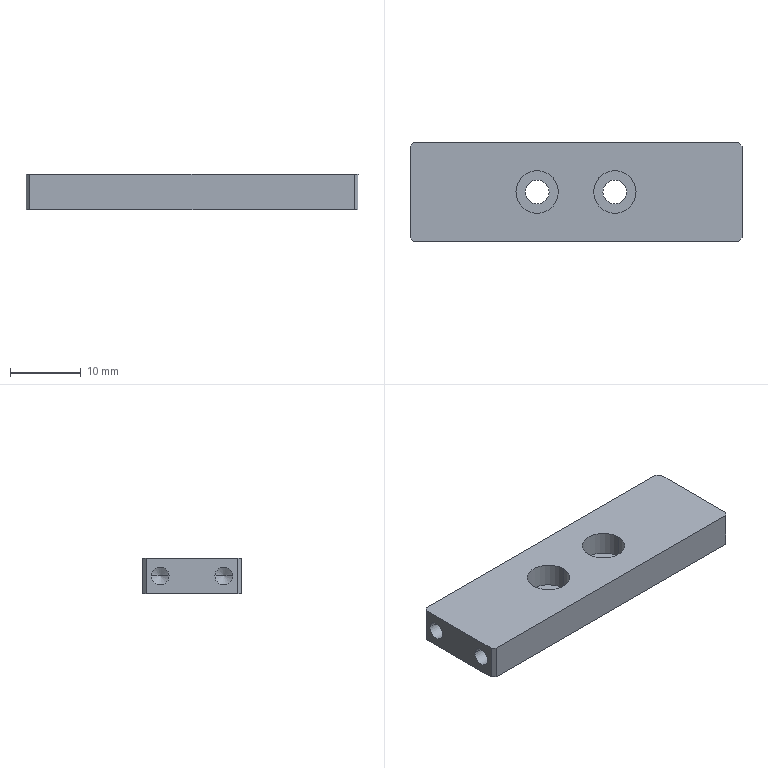Component | SolidWorks | F01AE00111-A5207-1 | 1 solid | 36 faces | box 47 x 14 x 5 mm | volume 2924 mm3 | cylinder 16 | plane 12 | cone 8 | commonest cylinder face diameters 2.5 x8 6 x4 3.4 x4
build123d program:
from build123d import *

# Parameters (mm, degrees)
SKETCH2_W                                            = 14
SKETCH2_H                                            = 5
BOSS_EXTRUDE1_DEPTH                                  = 23.5
HOLE_SIZE_ACCORDING_TO_THE_TYPE_OF_HEXAG_D           = 3.4
HOLE_SIZE_ACCORDING_TO_THE_TYPE_OF_HEXAG_CBORE_D     = 6
HOLE_SIZE_ACCORDING_TO_THE_TYPE_OF_HEXAG_CBORE_DEPTH = 3.4
M3_TAPPED_HOLE1_AT_2_COUNT                           = 2
M3_TAPPED_HOLE1_AT_2_PITCH                           = 9
CHAMFER1_SIZE                                        = 0.5


with BuildPart() as part:
    # Sketch2 → Boss-Extrude1 (new, symmetric)
    with BuildSketch(Plane.XY):
        with Locations((-7, 2.5)):
            Rectangle(SKETCH2_W, SKETCH2_H)
    extrude(amount=BOSS_EXTRUDE1_DEPTH, both=True)

    # Hole size according to the type of hexag (through all)
    with Locations(Plane(origin=(0, 5, 0), x_dir=(1, 0, 0), z_dir=(0, 1, 0))):
        with Locations((-7, 5.5), (-7, -5.5)):
            CounterBoreHole(HOLE_SIZE_ACCORDING_TO_THE_TYPE_OF_HEXAG_D / 2, HOLE_SIZE_ACCORDING_TO_THE_TYPE_OF_HEXAG_CBORE_D / 2, HOLE_SIZE_ACCORDING_TO_THE_TYPE_OF_HEXAG_CBORE_DEPTH)

    # Sketch7 → M3 Tapped Hole1 (revolve, cut)
    with BuildSketch(Plane(origin=(-2.5, 2.5, 23.5), x_dir=(0, -1, 0), z_dir=(1, 0, 0))):
        Polygon((0, 0), (0, 7.751), (1.25, 7), (1.25, 0), align=None)
    m3_tapped_hole1 = revolve(axis=Axis((-2.5, 2.5, 29.85), (0, 0, -1)), mode=Mode.SUBTRACT)

    # M3 Tapped Hole1 at 2: M3 Tapped Hole1 ×2
    with Locations(*[(-i * M3_TAPPED_HOLE1_AT_2_PITCH, 0, 0) for i in range(1, M3_TAPPED_HOLE1_AT_2_COUNT)]):
        add(m3_tapped_hole1, mode=Mode.SUBTRACT)

    # Mirror1: M3 Tapped Hole1 across plane
    add(m3_tapped_hole1.mirror(Plane.XY), mode=Mode.SUBTRACT)

    # Mirror1 copy 1 sketch → Mirror1 copy 1 (revolve, cut)
    with BuildSketch(Plane(origin=(-11.5, 2.5, -23.5), x_dir=(0, -1, 0), z_dir=(1, 0, 0))):
        Polygon((0, 0), (0, -7.751), (1.25, -7), (1.25, 0), align=None)
    revolve(axis=Axis((-11.5, 2.5, -29.85), (0, 0, -1)), mode=Mode.SUBTRACT)

    # Chamfer1
    chamfer1_edges = [part.edges().sort_by_distance(p)[0] for p in [
        (-14, 2.5, 23.5),
        (0, 2.5, 23.5),
        (-14, 2.5, -23.5),
        (0, 2.5, -23.5),
    ]]
    chamfer(chamfer1_edges, length=CHAMFER1_SIZE)


solid = part.part

# Placed as in the assembly
solid = solid.moved(Location((-17.181, -124.273, -285.979), (90, -90, 0)))
STEP:
#1=COLOUR_RGB('',0.7922,0.8196,0.9333);
#2=FILL_AREA_STYLE_COLOUR('',#1);
#3=FILL_AREA_STYLE('',(#2));
#4=SURFACE_STYLE_FILL_AREA(#3);
#5=SURFACE_SIDE_STYLE('',(#4));
#6=SURFACE_STYLE_USAGE(.BOTH.,#5);
#7=PRESENTATION_STYLE_ASSIGNMENT((#6));
#8=CARTESIAN_POINT('',(-0.0268,-4.489,-11.161));
#9=VERTEX_POINT('',#8);
#10=CARTESIAN_POINT('',(-0.0268,-4.391,-11.161));
#11=VERTEX_POINT('',#10);
#12=CARTESIAN_POINT('',(-0.0268,-4.44,-11.161));
#13=DIRECTION('',(1.,-0.,-0.));
#14=DIRECTION('',(0.,1.,0.));
#15=AXIS2_PLACEMENT_3D('',#12,#13,#14);
#16=CIRCLE('',#15,0.04921);
#17=EDGE_CURVE('',#9,#11,#16,.T.);
#18=ORIENTED_EDGE('',*,*,#17,.F.);
#19=CARTESIAN_POINT('',(0.2488,-4.489,-11.161));
#20=VERTEX_POINT('',#19);
#21=CARTESIAN_POINT('',(0.2488,-4.489,-11.161));
#22=DIRECTION('',(1.,-0.,-0.));
#23=VECTOR('',#22,39.37);
#24=LINE('',#21,#23);
#25=EDGE_CURVE('',#9,#20,#24,.T.);
#26=ORIENTED_EDGE('',*,*,#25,.T.);
#27=CARTESIAN_POINT('',(0.2488,-4.391,-11.161));
#28=VERTEX_POINT('',#27);
#29=CARTESIAN_POINT('',(0.2488,-4.44,-11.161));
#30=DIRECTION('',(1.,-0.,-0.));
#31=DIRECTION('',(0.,1.,0.));
#32=AXIS2_PLACEMENT_3D('',#29,#30,#31);
#33=CIRCLE('',#32,0.04921);
#34=EDGE_CURVE('',#20,#28,#33,.T.);
#35=ORIENTED_EDGE('',*,*,#34,.T.);
#36=CARTESIAN_POINT('',(0.2488,-4.391,-11.161));
#37=DIRECTION('',(1.,-0.,-0.));
#38=VECTOR('',#37,39.37);
#39=LINE('',#36,#38);
#40=EDGE_CURVE('',#11,#28,#39,.T.);
#41=ORIENTED_EDGE('',*,*,#40,.F.);
#42=EDGE_LOOP('',(#18,#26,#35,#41));
#43=FACE_OUTER_BOUND('',#42,.T.);
#44=CARTESIAN_POINT('',(0.2488,-4.44,-11.161));
#45=DIRECTION('',(1.,-0.,-0.));
#46=DIRECTION('',(0.,1.,0.));
#47=AXIS2_PLACEMENT_3D('',#44,#45,#46);
#48=CYLINDRICAL_SURFACE('',#47,0.04921);
#49=ADVANCED_FACE('',(#43),#48,.F.);
#50=CARTESIAN_POINT('',(-0.05637,-4.44,-11.161));
#51=VERTEX_POINT('',#50);
#52=CARTESIAN_POINT('',(-0.0268,-4.391,-11.161));
#53=DIRECTION('',(0.515,0.8572,-0.));
#54=VECTOR('',#53,39.37);
#55=LINE('',#52,#54);
#56=EDGE_CURVE('',#51,#11,#55,.T.);
#57=ORIENTED_EDGE('',*,*,#56,.F.);
#58=CARTESIAN_POINT('',(-0.0268,-4.489,-11.161));
#59=DIRECTION('',(0.515,-0.8572,-0.));
#60=VECTOR('',#59,39.37);
#61=LINE('',#58,#60);
#62=EDGE_CURVE('',#51,#9,#61,.T.);
#63=ORIENTED_EDGE('',*,*,#62,.T.);
#64=ORIENTED_EDGE('',*,*,#17,.T.);
#65=EDGE_LOOP('',(#57,#63,#64));
#66=FACE_OUTER_BOUND('',#65,.T.);
#67=CARTESIAN_POINT('',(-0.0268,-4.44,-11.161));
#68=DIRECTION('',(1.,-0.,-0.));
#69=DIRECTION('',(0.,1.,0.));
#70=AXIS2_PLACEMENT_3D('',#67,#68,#69);
#71=CONICAL_SURFACE('',#70,0.04921,1.03);
#72=ADVANCED_FACE('',(#66),#71,.F.);
#73=CARTESIAN_POINT('',(-0.0268,-4.843,-11.161));
#74=VERTEX_POINT('',#73);
#75=CARTESIAN_POINT('',(-0.0268,-4.745,-11.161));
#76=VERTEX_POINT('',#75);
#77=CARTESIAN_POINT('',(-0.0268,-4.794,-11.161));
#78=DIRECTION('',(1.,-0.,-0.));
#79=DIRECTION('',(0.,1.,0.));
#80=AXIS2_PLACEMENT_3D('',#77,#78,#79);
#81=CIRCLE('',#80,0.04921);
#82=EDGE_CURVE('',#74,#76,#81,.T.);
#83=ORIENTED_EDGE('',*,*,#82,.F.);
#84=CARTESIAN_POINT('',(0.2488,-4.843,-11.161));
#85=VERTEX_POINT('',#84);
#86=CARTESIAN_POINT('',(0.2488,-4.843,-11.161));
#87=DIRECTION('',(1.,-0.,-0.));
#88=VECTOR('',#87,39.37);
#89=LINE('',#86,#88);
#90=EDGE_CURVE('',#74,#85,#89,.T.);
#91=ORIENTED_EDGE('',*,*,#90,.T.);
#92=CARTESIAN_POINT('',(0.2488,-4.745,-11.161));
#93=VERTEX_POINT('',#92);
#94=CARTESIAN_POINT('',(0.2488,-4.794,-11.161));
#95=DIRECTION('',(1.,-0.,-0.));
#96=DIRECTION('',(0.,1.,0.));
#97=AXIS2_PLACEMENT_3D('',#94,#95,#96);
#98=CIRCLE('',#97,0.04921);
#99=EDGE_CURVE('',#85,#93,#98,.T.);
#100=ORIENTED_EDGE('',*,*,#99,.T.);
#101=CARTESIAN_POINT('',(0.2488,-4.745,-11.161));
#102=DIRECTION('',(1.,-0.,-0.));
#103=VECTOR('',#102,39.37);
#104=LINE('',#101,#103);
#105=EDGE_CURVE('',#76,#93,#104,.T.);
#106=ORIENTED_EDGE('',*,*,#105,.F.);
#107=EDGE_LOOP('',(#83,#91,#100,#106));
#108=FACE_OUTER_BOUND('',#107,.T.);
#109=CARTESIAN_POINT('',(0.2488,-4.794,-11.161));
#110=DIRECTION('',(1.,-0.,-0.));
#111=DIRECTION('',(0.,1.,0.));
#112=AXIS2_PLACEMENT_3D('',#109,#110,#111);
#113=CYLINDRICAL_SURFACE('',#112,0.04921);
#114=ADVANCED_FACE('',(#108),#113,.F.);
#115=CARTESIAN_POINT('',(-0.05637,-4.794,-11.161));
#116=VERTEX_POINT('',#115);
#117=CARTESIAN_POINT('',(-0.0268,-4.745,-11.161));
#118=DIRECTION('',(0.515,0.8572,-0.));
#119=VECTOR('',#118,39.37);
#120=LINE('',#117,#119);
#121=EDGE_CURVE('',#116,#76,#120,.T.);
#122=ORIENTED_EDGE('',*,*,#121,.F.);
#123=CARTESIAN_POINT('',(-0.0268,-4.843,-11.161));
#124=DIRECTION('',(0.515,-0.8572,-0.));
#125=VECTOR('',#124,39.37);
#126=LINE('',#123,#125);
#127=EDGE_CURVE('',#116,#74,#126,.T.);
#128=ORIENTED_EDGE('',*,*,#127,.T.);
#129=ORIENTED_EDGE('',*,*,#82,.T.);
#130=EDGE_LOOP('',(#122,#128,#129));
#131=FACE_OUTER_BOUND('',#130,.T.);
#132=CARTESIAN_POINT('',(-0.0268,-4.794,-11.161));
#133=DIRECTION('',(1.,-0.,-0.));
#134=DIRECTION('',(0.,1.,0.));
#135=AXIS2_PLACEMENT_3D('',#132,#133,#134);
#136=CONICAL_SURFACE('',#135,0.04921,1.03);
#137=ADVANCED_FACE('',(#131),#136,.F.);
#138=CARTESIAN_POINT('',(-1.326,-4.391,-11.161));
#139=VERTEX_POINT('',#138);
#140=CARTESIAN_POINT('',(-1.326,-4.489,-11.161));
#141=VERTEX_POINT('',#140);
#142=CARTESIAN_POINT('',(-1.326,-4.44,-11.161));
#143=DIRECTION('',(-1.,0.,0.));
#144=DIRECTION('',(0.,-1.,0.));
#145=AXIS2_PLACEMENT_3D('',#142,#143,#144);
#146=CIRCLE('',#145,0.04921);
#147=EDGE_CURVE('',#139,#141,#146,.T.);
#148=ORIENTED_EDGE('',*,*,#147,.F.);
#149=CARTESIAN_POINT('',(-1.602,-4.391,-11.161));
#150=VERTEX_POINT('',#149);
#151=CARTESIAN_POINT('',(-1.602,-4.391,-11.161));
#152=DIRECTION('',(-1.,0.,0.));
#153=VECTOR('',#152,39.37);
#154=LINE('',#151,#153);
#155=EDGE_CURVE('',#139,#150,#154,.T.);
#156=ORIENTED_EDGE('',*,*,#155,.T.);
#157=CARTESIAN_POINT('',(-1.602,-4.489,-11.161));
#158=VERTEX_POINT('',#157);
#159=CARTESIAN_POINT('',(-1.602,-4.44,-11.161));
#160=DIRECTION('',(-1.,0.,0.));
#161=DIRECTION('',(0.,-1.,0.));
#162=AXIS2_PLACEMENT_3D('',#159,#160,#161);
#163=CIRCLE('',#162,0.04921);
#164=EDGE_CURVE('',#150,#158,#163,.T.);
#165=ORIENTED_EDGE('',*,*,#164,.T.);
#166=CARTESIAN_POINT('',(-1.602,-4.489,-11.161));
#167=DIRECTION('',(-1.,0.,0.));
#168=VECTOR('',#167,39.37);
#169=LINE('',#166,#168);
#170=EDGE_CURVE('',#141,#158,#169,.T.);
#171=ORIENTED_EDGE('',*,*,#170,.F.);
#172=EDGE_LOOP('',(#148,#156,#165,#171));
#173=FACE_OUTER_BOUND('',#172,.T.);
#174=CARTESIAN_POINT('',(-1.602,-4.44,-11.161));
#175=DIRECTION('',(-1.,0.,0.));
#176=DIRECTION('',(0.,-1.,0.));
#177=AXIS2_PLACEMENT_3D('',#174,#175,#176);
#178=CYLINDRICAL_SURFACE('',#177,0.04921);
#179=ADVANCED_FACE('',(#173),#178,.F.);
#180=CARTESIAN_POINT('',(-1.296,-4.44,-11.161));
#181=VERTEX_POINT('',#180);
#182=CARTESIAN_POINT('',(-1.326,-4.489,-11.161));
#183=DIRECTION('',(-0.515,-0.8572,0.));
#184=VECTOR('',#183,39.37);
#185=LINE('',#182,#184);
#186=EDGE_CURVE('',#181,#141,#185,.T.);
#187=ORIENTED_EDGE('',*,*,#186,.F.);
#188=CARTESIAN_POINT('',(-1.326,-4.391,-11.161));
#189=DIRECTION('',(-0.515,0.8572,0.));
#190=VECTOR('',#189,39.37);
#191=LINE('',#188,#190);
#192=EDGE_CURVE('',#181,#139,#191,.T.);
#193=ORIENTED_EDGE('',*,*,#192,.T.);
#194=ORIENTED_EDGE('',*,*,#147,.T.);
#195=EDGE_LOOP('',(#187,#193,#194));
#196=FACE_OUTER_BOUND('',#195,.T.);
#197=CARTESIAN_POINT('',(-1.326,-4.44,-11.161));
#198=DIRECTION('',(-1.,0.,0.));
#199=DIRECTION('',(0.,-1.,0.));
#200=AXIS2_PLACEMENT_3D('',#197,#198,#199);
#201=CONICAL_SURFACE('',#200,0.04921,1.03);
#202=ADVANCED_FACE('',(#196),#201,.F.);
#203=CARTESIAN_POINT('',(-1.326,-4.745,-11.161));
#204=VERTEX_POINT('',#203);
#205=CARTESIAN_POINT('',(-1.326,-4.843,-11.161));
#206=VERTEX_POINT('',#205);
#207=CARTESIAN_POINT('',(-1.326,-4.794,-11.161));
#208=DIRECTION('',(-1.,0.,0.));
#209=DIRECTION('',(0.,-1.,0.));
#210=AXIS2_PLACEMENT_3D('',#207,#208,#209);
#211=CIRCLE('',#210,0.04921);
#212=EDGE_CURVE('',#204,#206,#211,.T.);
#213=ORIENTED_EDGE('',*,*,#212,.F.);
#214=CARTESIAN_POINT('',(-1.602,-4.745,-11.161));
#215=VERTEX_POINT('',#214);
#216=CARTESIAN_POINT('',(-1.602,-4.745,-11.161));
#217=DIRECTION('',(-1.,0.,0.));
#218=VECTOR('',#217,39.37);
#219=LINE('',#216,#218);
#220=EDGE_CURVE('',#204,#215,#219,.T.);
#221=ORIENTED_EDGE('',*,*,#220,.T.);
#222=CARTESIAN_POINT('',(-1.602,-4.843,-11.161));
#223=VERTEX_POINT('',#222);
#224=CARTESIAN_POINT('',(-1.602,-4.794,-11.161));
#225=DIRECTION('',(-1.,0.,0.));
#226=DIRECTION('',(0.,-1.,0.));
#227=AXIS2_PLACEMENT_3D('',#224,#225,#226);
#228=CIRCLE('',#227,0.04921);
#229=EDGE_CURVE('',#215,#223,#228,.T.);
#230=ORIENTED_EDGE('',*,*,#229,.T.);
#231=CARTESIAN_POINT('',(-1.602,-4.843,-11.161));
#232=DIRECTION('',(-1.,0.,0.));
#233=VECTOR('',#232,39.37);
#234=LINE('',#231,#233);
#235=EDGE_CURVE('',#206,#223,#234,.T.);
#236=ORIENTED_EDGE('',*,*,#235,.F.);
#237=EDGE_LOOP('',(#213,#221,#230,#236));
#238=FACE_OUTER_BOUND('',#237,.T.);
#239=CARTESIAN_POINT('',(-1.602,-4.794,-11.161));
#240=DIRECTION('',(-1.,0.,0.));
#241=DIRECTION('',(0.,-1.,0.));
#242=AXIS2_PLACEMENT_3D('',#239,#240,#241);
#243=CYLINDRICAL_SURFACE('',#242,0.04921);
#244=ADVANCED_FACE('',(#238),#243,.F.);
#245=CARTESIAN_POINT('',(-1.296,-4.794,-11.161));
#246=VERTEX_POINT('',#245);
#247=CARTESIAN_POINT('',(-1.326,-4.843,-11.161));
#248=DIRECTION('',(-0.515,-0.8572,0.));
#249=VECTOR('',#248,39.37);
#250=LINE('',#247,#249);
#251=EDGE_CURVE('',#246,#206,#250,.T.);
#252=ORIENTED_EDGE('',*,*,#251,.F.);
#253=CARTESIAN_POINT('',(-1.326,-4.745,-11.161));
#254=DIRECTION('',(-0.515,0.8572,0.));
#255=VECTOR('',#254,39.37);
#256=LINE('',#253,#255);
#257=EDGE_CURVE('',#246,#204,#256,.T.);
#258=ORIENTED_EDGE('',*,*,#257,.T.);
#259=ORIENTED_EDGE('',*,*,#212,.T.);
#260=EDGE_LOOP('',(#252,#258,#259));
#261=FACE_OUTER_BOUND('',#260,.T.);
#262=CARTESIAN_POINT('',(-1.326,-4.794,-11.161));
#263=DIRECTION('',(-1.,0.,0.));
#264=DIRECTION('',(0.,-1.,0.));
#265=AXIS2_PLACEMENT_3D('',#262,#263,#264);
#266=CONICAL_SURFACE('',#265,0.04921,1.03);
#267=ADVANCED_FACE('',(#261),#266,.F.);
#268=CARTESIAN_POINT('',(-0.3418,-4.617,-11.196));
#269=VERTEX_POINT('',#268);
#270=CARTESIAN_POINT('',(-0.578,-4.617,-11.196));
#271=VERTEX_POINT('',#270);
#272=CARTESIAN_POINT('',(-0.4599,-4.617,-11.196));
#273=DIRECTION('',(0.,-0.,1.));
#274=DIRECTION('',(-1.,0.,0.));
#275=AXIS2_PLACEMENT_3D('',#272,#273,#274);
#276=CIRCLE('',#275,0.1181);
#277=EDGE_CURVE('',#269,#271,#276,.T.);
#278=ORIENTED_EDGE('',*,*,#277,.F.);
#279=CARTESIAN_POINT('',(-0.3418,-4.617,-11.062));
#280=VERTEX_POINT('',#279);
#281=CARTESIAN_POINT('',(-0.3418,-4.617,-11.062));
#282=DIRECTION('',(0.,-0.,1.));
#283=VECTOR('',#282,39.37);
#284=LINE('',#281,#283);
#285=EDGE_CURVE('',#269,#280,#284,.T.);
#286=ORIENTED_EDGE('',*,*,#285,.T.);
#287=CARTESIAN_POINT('',(-0.578,-4.617,-11.062));
#288=VERTEX_POINT('',#287);
#289=CARTESIAN_POINT('',(-0.4599,-4.617,-11.062));
#290=DIRECTION('',(0.,-0.,1.));
#291=DIRECTION('',(-1.,0.,0.));
#292=AXIS2_PLACEMENT_3D('',#289,#290,#291);
#293=CIRCLE('',#292,0.1181);
#294=EDGE_CURVE('',#280,#288,#293,.T.);
#295=ORIENTED_EDGE('',*,*,#294,.T.);
#296=CARTESIAN_POINT('',(-0.578,-4.617,-11.062));
#297=DIRECTION('',(0.,-0.,1.));
#298=VECTOR('',#297,39.37);
#299=LINE('',#296,#298);
#300=EDGE_CURVE('',#271,#288,#299,.T.);
#301=ORIENTED_EDGE('',*,*,#300,.F.);
#302=EDGE_LOOP('',(#278,#286,#295,#301));
#303=FACE_OUTER_BOUND('',#302,.T.);
#304=CARTESIAN_POINT('',(-0.4599,-4.617,-11.062));
#305=DIRECTION('',(0.,-0.,1.));
#306=DIRECTION('',(-1.,0.,0.));
#307=AXIS2_PLACEMENT_3D('',#304,#305,#306);
#308=CYLINDRICAL_SURFACE('',#307,0.1181);
#309=ADVANCED_FACE('',(#303),#308,.F.);
#310=CARTESIAN_POINT('',(-0.3929,-4.617,-11.259));
#311=VERTEX_POINT('',#310);
#312=CARTESIAN_POINT('',(-0.5268,-4.617,-11.259));
#313=VERTEX_POINT('',#312);
#314=CARTESIAN_POINT('',(-0.4599,-4.617,-11.259));
#315=DIRECTION('',(0.,-0.,1.));
#316=DIRECTION('',(-1.,0.,0.));
#317=AXIS2_PLACEMENT_3D('',#314,#315,#316);
#318=CIRCLE('',#317,0.06693);
#319=EDGE_CURVE('',#311,#313,#318,.T.);
#320=ORIENTED_EDGE('',*,*,#319,.F.);
#321=CARTESIAN_POINT('',(-0.3929,-4.617,-11.196));
#322=VERTEX_POINT('',#321);
#323=CARTESIAN_POINT('',(-0.3929,-4.617,-11.062));
#324=DIRECTION('',(0.,-0.,1.));
#325=VECTOR('',#324,39.37);
#326=LINE('',#323,#325);
#327=EDGE_CURVE('',#311,#322,#326,.T.);
#328=ORIENTED_EDGE('',*,*,#327,.T.);
#329=CARTESIAN_POINT('',(-0.5268,-4.617,-11.196));
#330=VERTEX_POINT('',#329);
#331=CARTESIAN_POINT('',(-0.4599,-4.617,-11.196));
#332=DIRECTION('',(0.,-0.,1.));
#333=DIRECTION('',(-1.,0.,0.));
#334=AXIS2_PLACEMENT_3D('',#331,#332,#333);
#335=CIRCLE('',#334,0.06693);
#336=EDGE_CURVE('',#322,#330,#335,.T.);
#337=ORIENTED_EDGE('',*,*,#336,.T.);
#338=CARTESIAN_POINT('',(-0.5268,-4.617,-11.062));
#339=DIRECTION('',(0.,-0.,1.));
#340=VECTOR('',#339,39.37);
#341=LINE('',#338,#340);
#342=EDGE_CURVE('',#313,#330,#341,.T.);
#343=ORIENTED_EDGE('',*,*,#342,.F.);
#344=EDGE_LOOP('',(#320,#328,#337,#343));
#345=FACE_OUTER_BOUND('',#344,.T.);
#346=CARTESIAN_POINT('',(-0.4599,-4.617,-11.062));
#347=DIRECTION('',(0.,-0.,1.));
#348=DIRECTION('',(-1.,0.,0.));
#349=AXIS2_PLACEMENT_3D('',#346,#347,#348);
#350=CYLINDRICAL_SURFACE('',#349,0.06693);
#351=ADVANCED_FACE('',(#345),#350,.F.);
#352=CARTESIAN_POINT('',(-0.7748,-4.617,-11.196));
#353=VERTEX_POINT('',#352);
#354=CARTESIAN_POINT('',(-1.011,-4.617,-11.196));
#355=VERTEX_POINT('',#354);
#356=CARTESIAN_POINT('',(-0.8929,-4.617,-11.196));
#357=DIRECTION('',(0.,-0.,1.));
#358=DIRECTION('',(-1.,0.,0.));
#359=AXIS2_PLACEMENT_3D('',#356,#357,#358);
#360=CIRCLE('',#359,0.1181);
#361=EDGE_CURVE('',#353,#355,#360,.T.);
#362=ORIENTED_EDGE('',*,*,#361,.F.);
#363=CARTESIAN_POINT('',(-0.7748,-4.617,-11.062));
#364=VERTEX_POINT('',#363);
#365=CARTESIAN_POINT('',(-0.7748,-4.617,-11.062));
#366=DIRECTION('',(0.,-0.,1.));
#367=VECTOR('',#366,39.37);
#368=LINE('',#365,#367);
#369=EDGE_CURVE('',#353,#364,#368,.T.);
#370=ORIENTED_EDGE('',*,*,#369,.T.);
#371=CARTESIAN_POINT('',(-1.011,-4.617,-11.062));
#372=VERTEX_POINT('',#371);
#373=CARTESIAN_POINT('',(-0.8929,-4.617,-11.062));
#374=DIRECTION('',(0.,-0.,1.));
#375=DIRECTION('',(-1.,0.,0.));
#376=AXIS2_PLACEMENT_3D('',#373,#374,#375);
#377=CIRCLE('',#376,0.1181);
#378=EDGE_CURVE('',#364,#372,#377,.T.);
#379=ORIENTED_EDGE('',*,*,#378,.T.);
#380=CARTESIAN_POINT('',(-1.011,-4.617,-11.062));
#381=DIRECTION('',(0.,-0.,1.));
#382=VECTOR('',#381,39.37);
#383=LINE('',#380,#382);
#384=EDGE_CURVE('',#355,#372,#383,.T.);
#385=ORIENTED_EDGE('',*,*,#384,.F.);
#386=EDGE_LOOP('',(#362,#370,#379,#385));
#387=FACE_OUTER_BOUND('',#386,.T.);
#388=CARTESIAN_POINT('',(-0.8929,-4.617,-11.062));
#389=DIRECTION('',(0.,-0.,1.));
#390=DIRECTION('',(-1.,0.,0.));
#391=AXIS2_PLACEMENT_3D('',#388,#389,#390);
#392=CYLINDRICAL_SURFACE('',#391,0.1181);
#393=ADVANCED_FACE('',(#387),#392,.F.);
#394=CARTESIAN_POINT('',(-0.826,-4.617,-11.259));
#395=VERTEX_POINT('',#394);
#396=CARTESIAN_POINT('',(-0.9599,-4.617,-11.259));
#397=VERTEX_POINT('',#396);
#398=CARTESIAN_POINT('',(-0.8929,-4.617,-11.259));
#399=DIRECTION('',(0.,-0.,1.));
#400=DIRECTION('',(-1.,0.,0.));
#401=AXIS2_PLACEMENT_3D('',#398,#399,#400);
#402=CIRCLE('',#401,0.06693);
#403=EDGE_CURVE('',#395,#397,#402,.T.);
#404=ORIENTED_EDGE('',*,*,#403,.F.);
#405=CARTESIAN_POINT('',(-0.826,-4.617,-11.196));
#406=VERTEX_POINT('',#405);
#407=CARTESIAN_POINT('',(-0.826,-4.617,-11.062));
#408=DIRECTION('',(0.,-0.,1.));
#409=VECTOR('',#408,39.37);
#410=LINE('',#407,#409);
#411=EDGE_CURVE('',#395,#406,#410,.T.);
#412=ORIENTED_EDGE('',*,*,#411,.T.);
#413=CARTESIAN_POINT('',(-0.9599,-4.617,-11.196));
#414=VERTEX_POINT('',#413);
#415=CARTESIAN_POINT('',(-0.8929,-4.617,-11.196));
#416=DIRECTION('',(0.,-0.,1.));
#417=DIRECTION('',(-1.,0.,0.));
#418=AXIS2_PLACEMENT_3D('',#415,#416,#417);
#419=CIRCLE('',#418,0.06693);
#420=EDGE_CURVE('',#406,#414,#419,.T.);
#421=ORIENTED_EDGE('',*,*,#420,.T.);
#422=CARTESIAN_POINT('',(-0.9599,-4.617,-11.062));
#423=DIRECTION('',(0.,-0.,1.));
#424=VECTOR('',#423,39.37);
#425=LINE('',#422,#424);
#426=EDGE_CURVE('',#397,#414,#425,.T.);
#427=ORIENTED_EDGE('',*,*,#426,.F.);
#428=EDGE_LOOP('',(#404,#412,#421,#427));
#429=FACE_OUTER_BOUND('',#428,.T.);
#430=CARTESIAN_POINT('',(-0.8929,-4.617,-11.062));
#431=DIRECTION('',(0.,-0.,1.));
#432=DIRECTION('',(-1.,0.,0.));
#433=AXIS2_PLACEMENT_3D('',#430,#431,#432);
#434=CYLINDRICAL_SURFACE('',#433,0.06693);
#435=ADVANCED_FACE('',(#429),#434,.F.);
#436=CARTESIAN_POINT('',(-1.582,-4.893,-11.259));
#437=VERTEX_POINT('',#436);
#438=CARTESIAN_POINT('',(0.2291,-4.893,-11.259));
#439=VERTEX_POINT('',#438);
#440=CARTESIAN_POINT('',(-1.602,-4.893,-11.259));
#441=DIRECTION('',(1.,-0.,-0.));
#442=VECTOR('',#441,39.37);
#443=LINE('',#440,#442);
#444=EDGE_CURVE('',#437,#439,#443,.T.);
#445=ORIENTED_EDGE('',*,*,#444,.T.);
#446=CARTESIAN_POINT('',(0.2291,-4.893,-11.062));
#447=VERTEX_POINT('',#446);
#448=CARTESIAN_POINT('',(0.2291,-4.893,-11.062));
#449=DIRECTION('',(0.,-0.,1.));
#450=VECTOR('',#449,39.37);
#451=LINE('',#448,#450);
#452=EDGE_CURVE('',#439,#447,#451,.T.);
#453=ORIENTED_EDGE('',*,*,#452,.T.);
#454=CARTESIAN_POINT('',(-1.582,-4.893,-11.062));
#455=VERTEX_POINT('',#454);
#456=CARTESIAN_POINT('',(-1.602,-4.893,-11.062));
#457=DIRECTION('',(1.,-0.,-0.));
#458=VECTOR('',#457,39.37);
#459=LINE('',#456,#458);
#460=EDGE_CURVE('',#455,#447,#459,.T.);
#461=ORIENTED_EDGE('',*,*,#460,.F.);
#462=CARTESIAN_POINT('',(-1.582,-4.893,-11.062));
#463=DIRECTION('',(-0.,0.,-1.));
#464=VECTOR('',#463,39.37);
#465=LINE('',#462,#464);
#466=EDGE_CURVE('',#455,#437,#465,.T.);
#467=ORIENTED_EDGE('',*,*,#466,.T.);
#468=EDGE_LOOP('',(#445,#453,#461,#467));
#469=FACE_OUTER_BOUND('',#468,.T.);
#470=CARTESIAN_POINT('',(-1.602,-4.893,-11.062));
#471=DIRECTION('',(0.,1.,0.));
#472=DIRECTION('',(-0.,0.,-1.));
#473=AXIS2_PLACEMENT_3D('',#470,#471,#472);
#474=PLANE('',#473);
#475=ADVANCED_FACE('',(#469),#474,.F.);
#476=CARTESIAN_POINT('',(-0.4599,-4.617,-11.062));
#477=DIRECTION('',(0.,-0.,1.));
#478=DIRECTION('',(-1.,0.,0.));
#479=AXIS2_PLACEMENT_3D('',#476,#477,#478);
#480=CIRCLE('',#479,0.1181);
#481=EDGE_CURVE('',#288,#280,#480,.T.);
#482=ORIENTED_EDGE('',*,*,#481,.F.);
#483=ORIENTED_EDGE('',*,*,#294,.F.);
#484=EDGE_LOOP('',(#482,#483));
#485=FACE_BOUND('',#484,.T.);
#486=CARTESIAN_POINT('',(-0.8929,-4.617,-11.062));
#487=DIRECTION('',(0.,-0.,1.));
#488=DIRECTION('',(-1.,0.,0.));
#489=AXIS2_PLACEMENT_3D('',#486,#487,#488);
#490=CIRCLE('',#489,0.1181);
#491=EDGE_CURVE('',#372,#364,#490,.T.);
#492=ORIENTED_EDGE('',*,*,#491,.F.);
#493=ORIENTED_EDGE('',*,*,#378,.F.);
#494=EDGE_LOOP('',(#492,#493));
#495=FACE_BOUND('',#494,.T.);
#496=CARTESIAN_POINT('',(0.2488,-4.873,-11.062));
#497=VERTEX_POINT('',#496);
#498=CARTESIAN_POINT('',(0.2488,-4.361,-11.062));
#499=VERTEX_POINT('',#498);
#500=CARTESIAN_POINT('',(0.2488,-4.341,-11.062));
#501=DIRECTION('',(0.,1.,0.));
#502=VECTOR('',#501,39.37);
#503=LINE('',#500,#502);
#504=EDGE_CURVE('',#497,#499,#503,.T.);
#505=ORIENTED_EDGE('',*,*,#504,.T.);
#506=CARTESIAN_POINT('',(0.2291,-4.341,-11.062));
#507=VERTEX_POINT('',#506);
#508=CARTESIAN_POINT('',(0.2291,-4.341,-11.062));
#509=DIRECTION('',(-0.7071,0.7071,0.));
#510=VECTOR('',#509,39.37);
#511=LINE('',#508,#510);
#512=EDGE_CURVE('',#499,#507,#511,.T.);
#513=ORIENTED_EDGE('',*,*,#512,.T.);
#514=CARTESIAN_POINT('',(-1.582,-4.341,-11.062));
#515=VERTEX_POINT('',#514);
#516=CARTESIAN_POINT('',(-1.602,-4.341,-11.062));
#517=DIRECTION('',(1.,-0.,-0.));
#518=VECTOR('',#517,39.37);
#519=LINE('',#516,#518);
#520=EDGE_CURVE('',#515,#507,#519,.T.);
#521=ORIENTED_EDGE('',*,*,#520,.F.);
#522=CARTESIAN_POINT('',(-1.602,-4.361,-11.062));
#523=VERTEX_POINT('',#522);
#524=CARTESIAN_POINT('',(-1.602,-4.361,-11.062));
#525=DIRECTION('',(-0.7071,-0.7071,0.));
#526=VECTOR('',#525,39.37);
#527=LINE('',#524,#526);
#528=EDGE_CURVE('',#515,#523,#527,.T.);
#529=ORIENTED_EDGE('',*,*,#528,.T.);
#530=CARTESIAN_POINT('',(-1.602,-4.873,-11.062));
#531=VERTEX_POINT('',#530);
#532=CARTESIAN_POINT('',(-1.602,-4.341,-11.062));
#533=DIRECTION('',(0.,1.,0.));
#534=VECTOR('',#533,39.37);
#535=LINE('',#532,#534);
#536=EDGE_CURVE('',#531,#523,#535,.T.);
#537=ORIENTED_EDGE('',*,*,#536,.F.);
#538=CARTESIAN_POINT('',(-1.602,-4.873,-11.062));
#539=DIRECTION('',(0.7071,-0.7071,-0.));
#540=VECTOR('',#539,39.37);
#541=LINE('',#538,#540);
#542=EDGE_CURVE('',#531,#455,#541,.T.);
#543=ORIENTED_EDGE('',*,*,#542,.T.);
#544=ORIENTED_EDGE('',*,*,#460,.T.);
#545=CARTESIAN_POINT('',(0.2291,-4.893,-11.062));
#546=DIRECTION('',(0.7071,0.7071,-0.));
#547=VECTOR('',#546,39.37);
#548=LINE('',#545,#547);
#549=EDGE_CURVE('',#447,#497,#548,.T.);
#550=ORIENTED_EDGE('',*,*,#549,.T.);
#551=EDGE_LOOP('',(#505,#513,#521,#529,#537,#543,#544,#550));
#552=FACE_OUTER_BOUND('',#551,.T.);
#553=CARTESIAN_POINT('',(-1.602,-4.341,-11.062));
#554=DIRECTION('',(-0.,0.,-1.));
#555=DIRECTION('',(1.,-0.,-0.));
#556=AXIS2_PLACEMENT_3D('',#553,#554,#555);
#557=PLANE('',#556);
#558=ADVANCED_FACE('',(#485,#495,#552),#557,.F.);
#559=ORIENTED_EDGE('',*,*,#520,.T.);
#560=CARTESIAN_POINT('',(0.2291,-4.341,-11.259));
#561=VERTEX_POINT('',#560);
#562=CARTESIAN_POINT('',(0.2291,-4.341,-11.259));
#563=DIRECTION('',(-0.,0.,-1.));
#564=VECTOR('',#563,39.37);
#565=LINE('',#562,#564);
#566=EDGE_CURVE('',#507,#561,#565,.T.);
#567=ORIENTED_EDGE('',*,*,#566,.T.);
#568=CARTESIAN_POINT('',(-1.582,-4.341,-11.259));
#569=VERTEX_POINT('',#568);
#570=CARTESIAN_POINT('',(-1.602,-4.341,-11.259));
#571=DIRECTION('',(1.,-0.,-0.));
#572=VECTOR('',#571,39.37);
#573=LINE('',#570,#572);
#574=EDGE_CURVE('',#569,#561,#573,.T.);
#575=ORIENTED_EDGE('',*,*,#574,.F.);
#576=CARTESIAN_POINT('',(-1.582,-4.341,-11.259));
#577=DIRECTION('',(0.,-0.,1.));
#578=VECTOR('',#577,39.37);
#579=LINE('',#576,#578);
#580=EDGE_CURVE('',#569,#515,#579,.T.);
#581=ORIENTED_EDGE('',*,*,#580,.T.);
#582=EDGE_LOOP('',(#559,#567,#575,#581));
#583=FACE_OUTER_BOUND('',#582,.T.);
#584=CARTESIAN_POINT('',(-1.602,-4.341,-11.259));
#585=DIRECTION('',(-0.,-1.,-0.));
#586=DIRECTION('',(1.,-0.,-0.));
#587=AXIS2_PLACEMENT_3D('',#584,#585,#586);
#588=PLANE('',#587);
#589=ADVANCED_FACE('',(#583),#588,.F.);
#590=CARTESIAN_POINT('',(-0.4599,-4.617,-11.259));
#591=DIRECTION('',(0.,-0.,1.));
#592=DIRECTION('',(-1.,0.,0.));
#593=AXIS2_PLACEMENT_3D('',#590,#591,#592);
#594=CIRCLE('',#593,0.06693);
#595=EDGE_CURVE('',#313,#311,#594,.T.);
#596=ORIENTED_EDGE('',*,*,#595,.T.);
#597=ORIENTED_EDGE('',*,*,#319,.T.);
#598=EDGE_LOOP('',(#596,#597));
#599=FACE_BOUND('',#598,.T.);
#600=CARTESIAN_POINT('',(-0.8929,-4.617,-11.259));
#601=DIRECTION('',(0.,-0.,1.));
#602=DIRECTION('',(-1.,0.,0.));
#603=AXIS2_PLACEMENT_3D('',#600,#601,#602);
#604=CIRCLE('',#603,0.06693);
#605=EDGE_CURVE('',#397,#395,#604,.T.);
#606=ORIENTED_EDGE('',*,*,#605,.T.);
#607=ORIENTED_EDGE('',*,*,#403,.T.);
#608=EDGE_LOOP('',(#606,#607));
#609=FACE_BOUND('',#608,.T.);
#610=ORIENTED_EDGE('',*,*,#574,.T.);
#611=CARTESIAN_POINT('',(0.2488,-4.361,-11.259));
#612=VERTEX_POINT('',#611);
#613=CARTESIAN_POINT('',(0.2291,-4.341,-11.259));
#614=DIRECTION('',(0.7071,-0.7071,-0.));
#615=VECTOR('',#614,39.37);
#616=LINE('',#613,#615);
#617=EDGE_CURVE('',#561,#612,#616,.T.);
#618=ORIENTED_EDGE('',*,*,#617,.T.);
#619=CARTESIAN_POINT('',(0.2488,-4.873,-11.259));
#620=VERTEX_POINT('',#619);
#621=CARTESIAN_POINT('',(0.2488,-4.893,-11.259));
#622=DIRECTION('',(-0.,-1.,0.));
#623=VECTOR('',#622,39.37);
#624=LINE('',#621,#623);
#625=EDGE_CURVE('',#612,#620,#624,.T.);
#626=ORIENTED_EDGE('',*,*,#625,.T.);
#627=CARTESIAN_POINT('',(0.2291,-4.893,-11.259));
#628=DIRECTION('',(-0.7071,-0.7071,0.));
#629=VECTOR('',#628,39.37);
#630=LINE('',#627,#629);
#631=EDGE_CURVE('',#620,#439,#630,.T.);
#632=ORIENTED_EDGE('',*,*,#631,.T.);
#633=ORIENTED_EDGE('',*,*,#444,.F.);
#634=CARTESIAN_POINT('',(-1.602,-4.873,-11.259));
#635=VERTEX_POINT('',#634);
#636=CARTESIAN_POINT('',(-1.602,-4.873,-11.259));
#637=DIRECTION('',(-0.7071,0.7071,0.));
#638=VECTOR('',#637,39.37);
#639=LINE('',#636,#638);
#640=EDGE_CURVE('',#437,#635,#639,.T.);
#641=ORIENTED_EDGE('',*,*,#640,.T.);
#642=CARTESIAN_POINT('',(-1.602,-4.361,-11.259));
#643=VERTEX_POINT('',#642);
#644=CARTESIAN_POINT('',(-1.602,-4.893,-11.259));
#645=DIRECTION('',(-0.,-1.,0.));
#646=VECTOR('',#645,39.37);
#647=LINE('',#644,#646);
#648=EDGE_CURVE('',#643,#635,#647,.T.);
#649=ORIENTED_EDGE('',*,*,#648,.F.);
#650=CARTESIAN_POINT('',(-1.602,-4.361,-11.259));
#651=DIRECTION('',(0.7071,0.7071,-0.));
#652=VECTOR('',#651,39.37);
#653=LINE('',#650,#652);
#654=EDGE_CURVE('',#643,#569,#653,.T.);
#655=ORIENTED_EDGE('',*,*,#654,.T.);
#656=EDGE_LOOP('',(#610,#618,#626,#632,#633,#641,#649,#655));
#657=FACE_OUTER_BOUND('',#656,.T.);
#658=CARTESIAN_POINT('',(-1.602,-4.893,-11.259));
#659=DIRECTION('',(0.,0.,1.));
#660=DIRECTION('',(0.,1.,-0.));
#661=AXIS2_PLACEMENT_3D('',#658,#659,#660);
#662=PLANE('',#661);
#663=ADVANCED_FACE('',(#599,#609,#657),#662,.F.);
#664=CARTESIAN_POINT('',(-1.602,-4.44,-11.161));
#665=DIRECTION('',(-1.,0.,0.));
#666=DIRECTION('',(0.,-1.,0.));
#667=AXIS2_PLACEMENT_3D('',#664,#665,#666);
#668=CIRCLE('',#667,0.04921);
#669=EDGE_CURVE('',#158,#150,#668,.T.);
#670=ORIENTED_EDGE('',*,*,#669,.F.);
#671=ORIENTED_EDGE('',*,*,#164,.F.);
#672=EDGE_LOOP('',(#670,#671));
#673=FACE_BOUND('',#672,.T.);
#674=CARTESIAN_POINT('',(-1.602,-4.794,-11.161));
#675=DIRECTION('',(-1.,0.,0.));
#676=DIRECTION('',(0.,-1.,0.));
#677=AXIS2_PLACEMENT_3D('',#674,#675,#676);
#678=CIRCLE('',#677,0.04921);
#679=EDGE_CURVE('',#223,#215,#678,.T.);
#680=ORIENTED_EDGE('',*,*,#679,.F.);
#681=ORIENTED_EDGE('',*,*,#229,.F.);
#682=EDGE_LOOP('',(#680,#681));
#683=FACE_BOUND('',#682,.T.);
#684=ORIENTED_EDGE('',*,*,#536,.T.);
#685=CARTESIAN_POINT('',(-1.602,-4.361,-11.259));
#686=DIRECTION('',(-0.,0.,-1.));
#687=VECTOR('',#686,39.37);
#688=LINE('',#685,#687);
#689=EDGE_CURVE('',#523,#643,#688,.T.);
#690=ORIENTED_EDGE('',*,*,#689,.T.);
#691=ORIENTED_EDGE('',*,*,#648,.T.);
#692=CARTESIAN_POINT('',(-1.602,-4.873,-11.259));
#693=DIRECTION('',(0.,-0.,1.));
#694=VECTOR('',#693,39.37);
#695=LINE('',#692,#694);
#696=EDGE_CURVE('',#635,#531,#695,.T.);
#697=ORIENTED_EDGE('',*,*,#696,.T.);
#698=EDGE_LOOP('',(#684,#690,#691,#697));
#699=FACE_OUTER_BOUND('',#698,.T.);
#700=CARTESIAN_POINT('',(-1.602,-4.893,-11.259));
#701=DIRECTION('',(1.,-0.,-0.));
#702=DIRECTION('',(0.,1.,0.));
#703=AXIS2_PLACEMENT_3D('',#700,#701,#702);
#704=PLANE('',#703);
#705=ADVANCED_FACE('',(#673,#683,#699),#704,.F.);
#706=CARTESIAN_POINT('',(0.2488,-4.44,-11.161));
#707=DIRECTION('',(1.,-0.,-0.));
#708=DIRECTION('',(0.,1.,0.));
#709=AXIS2_PLACEMENT_3D('',#706,#707,#708);
#710=CIRCLE('',#709,0.04921);
#711=EDGE_CURVE('',#28,#20,#710,.T.);
#712=ORIENTED_EDGE('',*,*,#711,.F.);
#713=ORIENTED_EDGE('',*,*,#34,.F.);
#714=EDGE_LOOP('',(#712,#713));
#715=FACE_BOUND('',#714,.T.);
#716=CARTESIAN_POINT('',(0.2488,-4.794,-11.161));
#717=DIRECTION('',(1.,-0.,-0.));
#718=DIRECTION('',(0.,1.,0.));
#719=AXIS2_PLACEMENT_3D('',#716,#717,#718);
#720=CIRCLE('',#719,0.04921);
#721=EDGE_CURVE('',#93,#85,#720,.T.);
#722=ORIENTED_EDGE('',*,*,#721,.F.);
#723=ORIENTED_EDGE('',*,*,#99,.F.);
#724=EDGE_LOOP('',(#722,#723));
#725=FACE_BOUND('',#724,.T.);
#726=ORIENTED_EDGE('',*,*,#625,.F.);
#727=CARTESIAN_POINT('',(0.2488,-4.361,-11.062));
#728=DIRECTION('',(0.,-0.,1.));
#729=VECTOR('',#728,39.37);
#730=LINE('',#727,#729);
#731=EDGE_CURVE('',#612,#499,#730,.T.);
#732=ORIENTED_EDGE('',*,*,#731,.T.);
#733=ORIENTED_EDGE('',*,*,#504,.F.);
#734=CARTESIAN_POINT('',(0.2488,-4.873,-11.259));
#735=DIRECTION('',(-0.,0.,-1.));
#736=VECTOR('',#735,39.37);
#737=LINE('',#734,#736);
#738=EDGE_CURVE('',#497,#620,#737,.T.);
#739=ORIENTED_EDGE('',*,*,#738,.T.);
#740=EDGE_LOOP('',(#726,#732,#733,#739));
#741=FACE_OUTER_BOUND('',#740,.T.);
#742=CARTESIAN_POINT('',(0.2488,-4.893,-11.259));
#743=DIRECTION('',(1.,-0.,-0.));
#744=DIRECTION('',(0.,1.,0.));
#745=AXIS2_PLACEMENT_3D('',#742,#743,#744);
#746=PLANE('',#745);
#747=ADVANCED_FACE('',(#715,#725,#741),#746,.T.);
#748=ORIENTED_EDGE('',*,*,#411,.F.);
#749=ORIENTED_EDGE('',*,*,#605,.F.);
#750=ORIENTED_EDGE('',*,*,#426,.T.);
#751=CARTESIAN_POINT('',(-0.8929,-4.617,-11.196));
#752=DIRECTION('',(0.,-0.,1.));
#753=DIRECTION('',(-1.,0.,0.));
#754=AXIS2_PLACEMENT_3D('',#751,#752,#753);
#755=CIRCLE('',#754,0.06693);
#756=EDGE_CURVE('',#414,#406,#755,.T.);
#757=ORIENTED_EDGE('',*,*,#756,.T.);
#758=EDGE_LOOP('',(#748,#749,#750,#757));
#759=FACE_OUTER_BOUND('',#758,.T.);
#760=CARTESIAN_POINT('',(-0.8929,-4.617,-11.062));
#761=DIRECTION('',(0.,-0.,1.));
#762=DIRECTION('',(-1.,0.,0.));
#763=AXIS2_PLACEMENT_3D('',#760,#761,#762);
#764=CYLINDRICAL_SURFACE('',#763,0.06693);
#765=ADVANCED_FACE('',(#759),#764,.F.);
#766=ORIENTED_EDGE('',*,*,#756,.F.);
#767=ORIENTED_EDGE('',*,*,#420,.F.);
#768=EDGE_LOOP('',(#766,#767));
#769=FACE_BOUND('',#768,.T.);
#770=CARTESIAN_POINT('',(-0.8929,-4.617,-11.196));
#771=DIRECTION('',(0.,-0.,1.));
#772=DIRECTION('',(-1.,0.,0.));
#773=AXIS2_PLACEMENT_3D('',#770,#771,#772);
#774=CIRCLE('',#773,0.1181);
#775=EDGE_CURVE('',#355,#353,#774,.T.);
#776=ORIENTED_EDGE('',*,*,#775,.T.);
#777=ORIENTED_EDGE('',*,*,#361,.T.);
#778=EDGE_LOOP('',(#776,#777));
#779=FACE_OUTER_BOUND('',#778,.T.);
#780=CARTESIAN_POINT('',(-0.8929,-4.684,-11.196));
#781=DIRECTION('',(-0.,0.,-1.));
#782=DIRECTION('',(1.,-0.,-0.));
#783=AXIS2_PLACEMENT_3D('',#780,#781,#782);
#784=PLANE('',#783);
#785=ADVANCED_FACE('',(#769,#779),#784,.F.);
#786=ORIENTED_EDGE('',*,*,#369,.F.);
#787=ORIENTED_EDGE('',*,*,#775,.F.);
#788=ORIENTED_EDGE('',*,*,#384,.T.);
#789=ORIENTED_EDGE('',*,*,#491,.T.);
#790=EDGE_LOOP('',(#786,#787,#788,#789));
#791=FACE_OUTER_BOUND('',#790,.T.);
#792=CARTESIAN_POINT('',(-0.8929,-4.617,-11.062));
#793=DIRECTION('',(0.,-0.,1.));
#794=DIRECTION('',(-1.,0.,0.));
#795=AXIS2_PLACEMENT_3D('',#792,#793,#794);
#796=CYLINDRICAL_SURFACE('',#795,0.1181);
#797=ADVANCED_FACE('',(#791),#796,.F.);
#798=ORIENTED_EDGE('',*,*,#327,.F.);
#799=ORIENTED_EDGE('',*,*,#595,.F.);
#800=ORIENTED_EDGE('',*,*,#342,.T.);
#801=CARTESIAN_POINT('',(-0.4599,-4.617,-11.196));
#802=DIRECTION('',(0.,-0.,1.));
#803=DIRECTION('',(-1.,0.,0.));
#804=AXIS2_PLACEMENT_3D('',#801,#802,#803);
#805=CIRCLE('',#804,0.06693);
#806=EDGE_CURVE('',#330,#322,#805,.T.);
#807=ORIENTED_EDGE('',*,*,#806,.T.);
#808=EDGE_LOOP('',(#798,#799,#800,#807));
#809=FACE_OUTER_BOUND('',#808,.T.);
#810=CARTESIAN_POINT('',(-0.4599,-4.617,-11.062));
#811=DIRECTION('',(0.,-0.,1.));
#812=DIRECTION('',(-1.,0.,0.));
#813=AXIS2_PLACEMENT_3D('',#810,#811,#812);
#814=CYLINDRICAL_SURFACE('',#813,0.06693);
#815=ADVANCED_FACE('',(#809),#814,.F.);
#816=ORIENTED_EDGE('',*,*,#806,.F.);
#817=ORIENTED_EDGE('',*,*,#336,.F.);
#818=EDGE_LOOP('',(#816,#817));
#819=FACE_BOUND('',#818,.T.);
#820=CARTESIAN_POINT('',(-0.4599,-4.617,-11.196));
#821=DIRECTION('',(0.,-0.,1.));
#822=DIRECTION('',(-1.,0.,0.));
#823=AXIS2_PLACEMENT_3D('',#820,#821,#822);
#824=CIRCLE('',#823,0.1181);
#825=EDGE_CURVE('',#271,#269,#824,.T.);
#826=ORIENTED_EDGE('',*,*,#825,.T.);
#827=ORIENTED_EDGE('',*,*,#277,.T.);
#828=EDGE_LOOP('',(#826,#827));
#829=FACE_OUTER_BOUND('',#828,.T.);
#830=CARTESIAN_POINT('',(-0.4599,-4.684,-11.196));
#831=DIRECTION('',(-0.,0.,-1.));
#832=DIRECTION('',(1.,-0.,-0.));
#833=AXIS2_PLACEMENT_3D('',#830,#831,#832);
#834=PLANE('',#833);
#835=ADVANCED_FACE('',(#819,#829),#834,.F.);
#836=ORIENTED_EDGE('',*,*,#285,.F.);
#837=ORIENTED_EDGE('',*,*,#825,.F.);
#838=ORIENTED_EDGE('',*,*,#300,.T.);
#839=ORIENTED_EDGE('',*,*,#481,.T.);
#840=EDGE_LOOP('',(#836,#837,#838,#839));
#841=FACE_OUTER_BOUND('',#840,.T.);
#842=CARTESIAN_POINT('',(-0.4599,-4.617,-11.062));
#843=DIRECTION('',(0.,-0.,1.));
#844=DIRECTION('',(-1.,0.,0.));
#845=AXIS2_PLACEMENT_3D('',#842,#843,#844);
#846=CYLINDRICAL_SURFACE('',#845,0.1181);
#847=ADVANCED_FACE('',(#841),#846,.F.);
#848=ORIENTED_EDGE('',*,*,#257,.F.);
#849=ORIENTED_EDGE('',*,*,#251,.T.);
#850=CARTESIAN_POINT('',(-1.326,-4.794,-11.161));
#851=DIRECTION('',(-1.,0.,0.));
#852=DIRECTION('',(0.,-1.,0.));
#853=AXIS2_PLACEMENT_3D('',#850,#851,#852);
#854=CIRCLE('',#853,0.04921);
#855=EDGE_CURVE('',#206,#204,#854,.T.);
#856=ORIENTED_EDGE('',*,*,#855,.T.);
#857=EDGE_LOOP('',(#848,#849,#856));
#858=FACE_OUTER_BOUND('',#857,.T.);
#859=CARTESIAN_POINT('',(-1.326,-4.794,-11.161));
#860=DIRECTION('',(-1.,0.,0.));
#861=DIRECTION('',(0.,-1.,0.));
#862=AXIS2_PLACEMENT_3D('',#859,#860,#861);
#863=CONICAL_SURFACE('',#862,0.04921,1.03);
#864=ADVANCED_FACE('',(#858),#863,.F.);
#865=ORIENTED_EDGE('',*,*,#220,.F.);
#866=ORIENTED_EDGE('',*,*,#855,.F.);
#867=ORIENTED_EDGE('',*,*,#235,.T.);
#868=ORIENTED_EDGE('',*,*,#679,.T.);
#869=EDGE_LOOP('',(#865,#866,#867,#868));
#870=FACE_OUTER_BOUND('',#869,.T.);
#871=CARTESIAN_POINT('',(-1.602,-4.794,-11.161));
#872=DIRECTION('',(-1.,0.,0.));
#873=DIRECTION('',(0.,-1.,0.));
#874=AXIS2_PLACEMENT_3D('',#871,#872,#873);
#875=CYLINDRICAL_SURFACE('',#874,0.04921);
#876=ADVANCED_FACE('',(#870),#875,.F.);
#877=ORIENTED_EDGE('',*,*,#192,.F.);
#878=ORIENTED_EDGE('',*,*,#186,.T.);
#879=CARTESIAN_POINT('',(-1.326,-4.44,-11.161));
#880=DIRECTION('',(-1.,0.,0.));
#881=DIRECTION('',(0.,-1.,0.));
#882=AXIS2_PLACEMENT_3D('',#879,#880,#881);
#883=CIRCLE('',#882,0.04921);
#884=EDGE_CURVE('',#141,#139,#883,.T.);
#885=ORIENTED_EDGE('',*,*,#884,.T.);
#886=EDGE_LOOP('',(#877,#878,#885));
#887=FACE_OUTER_BOUND('',#886,.T.);
#888=CARTESIAN_POINT('',(-1.326,-4.44,-11.161));
#889=DIRECTION('',(-1.,0.,0.));
#890=DIRECTION('',(0.,-1.,0.));
#891=AXIS2_PLACEMENT_3D('',#888,#889,#890);
#892=CONICAL_SURFACE('',#891,0.04921,1.03);
#893=ADVANCED_FACE('',(#887),#892,.F.);
#894=ORIENTED_EDGE('',*,*,#155,.F.);
#895=ORIENTED_EDGE('',*,*,#884,.F.);
#896=ORIENTED_EDGE('',*,*,#170,.T.);
#897=ORIENTED_EDGE('',*,*,#669,.T.);
#898=EDGE_LOOP('',(#894,#895,#896,#897));
#899=FACE_OUTER_BOUND('',#898,.T.);
#900=CARTESIAN_POINT('',(-1.602,-4.44,-11.161));
#901=DIRECTION('',(-1.,0.,0.));
#902=DIRECTION('',(0.,-1.,0.));
#903=AXIS2_PLACEMENT_3D('',#900,#901,#902);
#904=CYLINDRICAL_SURFACE('',#903,0.04921);
#905=ADVANCED_FACE('',(#899),#904,.F.);
#906=ORIENTED_EDGE('',*,*,#127,.F.);
#907=ORIENTED_EDGE('',*,*,#121,.T.);
#908=CARTESIAN_POINT('',(-0.0268,-4.794,-11.161));
#909=DIRECTION('',(1.,-0.,-0.));
#910=DIRECTION('',(0.,1.,0.));
#911=AXIS2_PLACEMENT_3D('',#908,#909,#910);
#912=CIRCLE('',#911,0.04921);
#913=EDGE_CURVE('',#76,#74,#912,.T.);
#914=ORIENTED_EDGE('',*,*,#913,.T.);
#915=EDGE_LOOP('',(#906,#907,#914));
#916=FACE_OUTER_BOUND('',#915,.T.);
#917=CARTESIAN_POINT('',(-0.0268,-4.794,-11.161));
#918=DIRECTION('',(1.,-0.,-0.));
#919=DIRECTION('',(0.,1.,0.));
#920=AXIS2_PLACEMENT_3D('',#917,#918,#919);
#921=CONICAL_SURFACE('',#920,0.04921,1.03);
#922=ADVANCED_FACE('',(#916),#921,.F.);
#923=ORIENTED_EDGE('',*,*,#90,.F.);
#924=ORIENTED_EDGE('',*,*,#913,.F.);
#925=ORIENTED_EDGE('',*,*,#105,.T.);
#926=ORIENTED_EDGE('',*,*,#721,.T.);
#927=EDGE_LOOP('',(#923,#924,#925,#926));
#928=FACE_OUTER_BOUND('',#927,.T.);
#929=CARTESIAN_POINT('',(0.2488,-4.794,-11.161));
#930=DIRECTION('',(1.,-0.,-0.));
#931=DIRECTION('',(0.,1.,0.));
#932=AXIS2_PLACEMENT_3D('',#929,#930,#931);
#933=CYLINDRICAL_SURFACE('',#932,0.04921);
#934=ADVANCED_FACE('',(#928),#933,.F.);
#935=ORIENTED_EDGE('',*,*,#62,.F.);
#936=ORIENTED_EDGE('',*,*,#56,.T.);
#937=CARTESIAN_POINT('',(-0.0268,-4.44,-11.161));
#938=DIRECTION('',(1.,-0.,-0.));
#939=DIRECTION('',(0.,1.,0.));
#940=AXIS2_PLACEMENT_3D('',#937,#938,#939);
#941=CIRCLE('',#940,0.04921);
#942=EDGE_CURVE('',#11,#9,#941,.T.);
#943=ORIENTED_EDGE('',*,*,#942,.T.);
#944=EDGE_LOOP('',(#935,#936,#943));
#945=FACE_OUTER_BOUND('',#944,.T.);
#946=CARTESIAN_POINT('',(-0.0268,-4.44,-11.161));
#947=DIRECTION('',(1.,-0.,-0.));
#948=DIRECTION('',(0.,1.,0.));
#949=AXIS2_PLACEMENT_3D('',#946,#947,#948);
#950=CONICAL_SURFACE('',#949,0.04921,1.03);
#951=ADVANCED_FACE('',(#945),#950,.F.);
#952=ORIENTED_EDGE('',*,*,#25,.F.);
#953=ORIENTED_EDGE('',*,*,#942,.F.);
#954=ORIENTED_EDGE('',*,*,#40,.T.);
#955=ORIENTED_EDGE('',*,*,#711,.T.);
#956=EDGE_LOOP('',(#952,#953,#954,#955));
#957=FACE_OUTER_BOUND('',#956,.T.);
#958=CARTESIAN_POINT('',(0.2488,-4.44,-11.161));
#959=DIRECTION('',(1.,-0.,-0.));
#960=DIRECTION('',(0.,1.,0.));
#961=AXIS2_PLACEMENT_3D('',#958,#959,#960);
#962=CYLINDRICAL_SURFACE('',#961,0.04921);
#963=ADVANCED_FACE('',(#957),#962,.F.);
#964=ORIENTED_EDGE('',*,*,#512,.F.);
#965=ORIENTED_EDGE('',*,*,#731,.F.);
#966=ORIENTED_EDGE('',*,*,#617,.F.);
#967=ORIENTED_EDGE('',*,*,#566,.F.);
#968=EDGE_LOOP('',(#964,#965,#966,#967));
#969=FACE_OUTER_BOUND('',#968,.T.);
#970=CARTESIAN_POINT('',(0.2291,-4.341,-11.259));
#971=DIRECTION('',(0.7071,0.7071,-0.));
#972=DIRECTION('',(0.,-0.,1.));
#973=AXIS2_PLACEMENT_3D('',#970,#971,#972);
#974=PLANE('',#973);
#975=ADVANCED_FACE('',(#969),#974,.T.);
#976=ORIENTED_EDGE('',*,*,#631,.F.);
#977=ORIENTED_EDGE('',*,*,#738,.F.);
#978=ORIENTED_EDGE('',*,*,#549,.F.);
#979=ORIENTED_EDGE('',*,*,#452,.F.);
#980=EDGE_LOOP('',(#976,#977,#978,#979));
#981=FACE_OUTER_BOUND('',#980,.T.);
#982=CARTESIAN_POINT('',(0.2291,-4.893,-11.062));
#983=DIRECTION('',(0.7071,-0.7071,-0.));
#984=DIRECTION('',(-0.,0.,-1.));
#985=AXIS2_PLACEMENT_3D('',#982,#983,#984);
#986=PLANE('',#985);
#987=ADVANCED_FACE('',(#981),#986,.T.);
#988=ORIENTED_EDGE('',*,*,#528,.F.);
#989=ORIENTED_EDGE('',*,*,#580,.F.);
#990=ORIENTED_EDGE('',*,*,#654,.F.);
#991=ORIENTED_EDGE('',*,*,#689,.F.);
#992=EDGE_LOOP('',(#988,#989,#990,#991));
#993=FACE_OUTER_BOUND('',#992,.T.);
#994=CARTESIAN_POINT('',(-1.602,-4.361,-11.259));
#995=DIRECTION('',(0.7071,-0.7071,-0.));
#996=DIRECTION('',(-0.,0.,-1.));
#997=AXIS2_PLACEMENT_3D('',#994,#995,#996);
#998=PLANE('',#997);
#999=ADVANCED_FACE('',(#993),#998,.F.);
#1000=ORIENTED_EDGE('',*,*,#640,.F.);
#1001=ORIENTED_EDGE('',*,*,#466,.F.);
#1002=ORIENTED_EDGE('',*,*,#542,.F.);
#1003=ORIENTED_EDGE('',*,*,#696,.F.);
#1004=EDGE_LOOP('',(#1000,#1001,#1002,#1003));
#1005=FACE_OUTER_BOUND('',#1004,.T.);
#1006=CARTESIAN_POINT('',(-1.602,-4.873,-11.259));
#1007=DIRECTION('',(0.7071,0.7071,-0.));
#1008=DIRECTION('',(0.,-0.,1.));
#1009=AXIS2_PLACEMENT_3D('',#1006,#1007,#1008);
#1010=PLANE('',#1009);
#1011=ADVANCED_FACE('',(#1005),#1010,.F.);
#1012=CLOSED_SHELL('',(#49,#72,#114,#137,#179,#202,#244,#267,#309,#351,#393,#435,#475,#558,#589,#663,#705,#747,#765,#785,#797,#815,#835,#847,#864,#876,#893,#905,#922,#934,#951,#963,#975,#987,#999,#1011));
#1013=MANIFOLD_SOLID_BREP('',#1012);
#1014=STYLED_ITEM('',(#7),#1013);
#1015=PRESENTATION_LAYER_ASSIGNMENT('','',(#1014));
#1016=CARTESIAN_POINT('',(0.,0.,0.));
#1017=DIRECTION('',(0.,0.,1.));
#1018=DIRECTION('',(1.,0.,0.));
#1019=AXIS2_PLACEMENT_3D('',#1016,#1017,#1018);
#1020=(LENGTH_UNIT()NAMED_UNIT(*)SI_UNIT($,.METRE.));
#1021=LENGTH_MEASURE_WITH_UNIT(LENGTH_MEASURE(0.0254),#1020);
#1022=DIMENSIONAL_EXPONENTS(1.,0.,0.,0.,0.,0.,0.);
#1023=(CONVERSION_BASED_UNIT('',#1021)LENGTH_UNIT()NAMED_UNIT(#1022));
#1024=UNCERTAINTY_MEASURE_WITH_UNIT(LENGTH_MEASURE(0.00001),#1023,'','');
#1025=(NAMED_UNIT(*)PLANE_ANGLE_UNIT()SI_UNIT($,.RADIAN.));
#1026=(NAMED_UNIT(*)SI_UNIT($,.STERADIAN.)SOLID_ANGLE_UNIT());
#1027=(GEOMETRIC_REPRESENTATION_CONTEXT(3)GLOBAL_UNCERTAINTY_ASSIGNED_CONTEXT((#1024))GLOBAL_UNIT_ASSIGNED_CONTEXT((#1023,#1025,#1026))REPRESENTATION_CONTEXT('',''));
#1028=ADVANCED_BREP_SHAPE_REPRESENTATION('',(#1013,#1019),#1027);
#1029=(LENGTH_UNIT()NAMED_UNIT(*)SI_UNIT($,.METRE.));
#1030=LENGTH_MEASURE_WITH_UNIT(LENGTH_MEASURE(0.0254),#1029);
#1031=DIMENSIONAL_EXPONENTS(1.,0.,0.,0.,0.,0.,0.);
#1032=(CONVERSION_BASED_UNIT('',#1030)LENGTH_UNIT()NAMED_UNIT(#1031));
#1033=UNCERTAINTY_MEASURE_WITH_UNIT(LENGTH_MEASURE(0.00001),#1032,'','');
#1034=(NAMED_UNIT(*)PLANE_ANGLE_UNIT()SI_UNIT($,.RADIAN.));
#1035=(NAMED_UNIT(*)SI_UNIT($,.STERADIAN.)SOLID_ANGLE_UNIT());
#1036=(GEOMETRIC_REPRESENTATION_CONTEXT(3)GLOBAL_UNCERTAINTY_ASSIGNED_CONTEXT((#1033))GLOBAL_UNIT_ASSIGNED_CONTEXT((#1032,#1034,#1035))REPRESENTATION_CONTEXT('',''));
#1037=MECHANICAL_DESIGN_GEOMETRIC_PRESENTATION_REPRESENTATION('',(#1014),#1036);